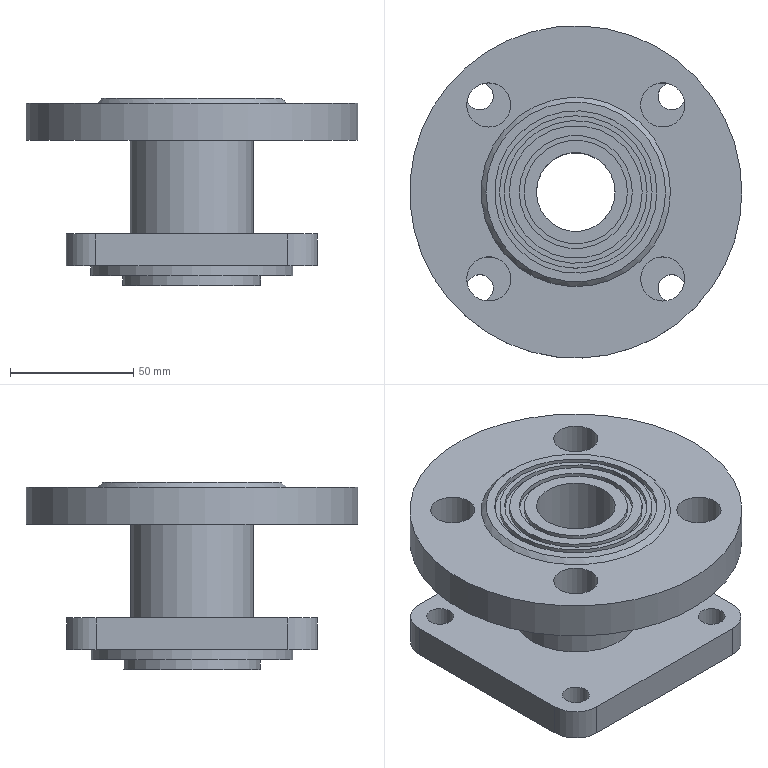Component | NX | VALVE_BONNET | 1 solid | 43 faces | volume 377577 mm3 | cylinder 24 | plane 18 | cone 1 | commonest cylinder face diameters 24 x4 11 x4 18 x4 82 x1 56 x1 50 x1 135 x1 32 x1